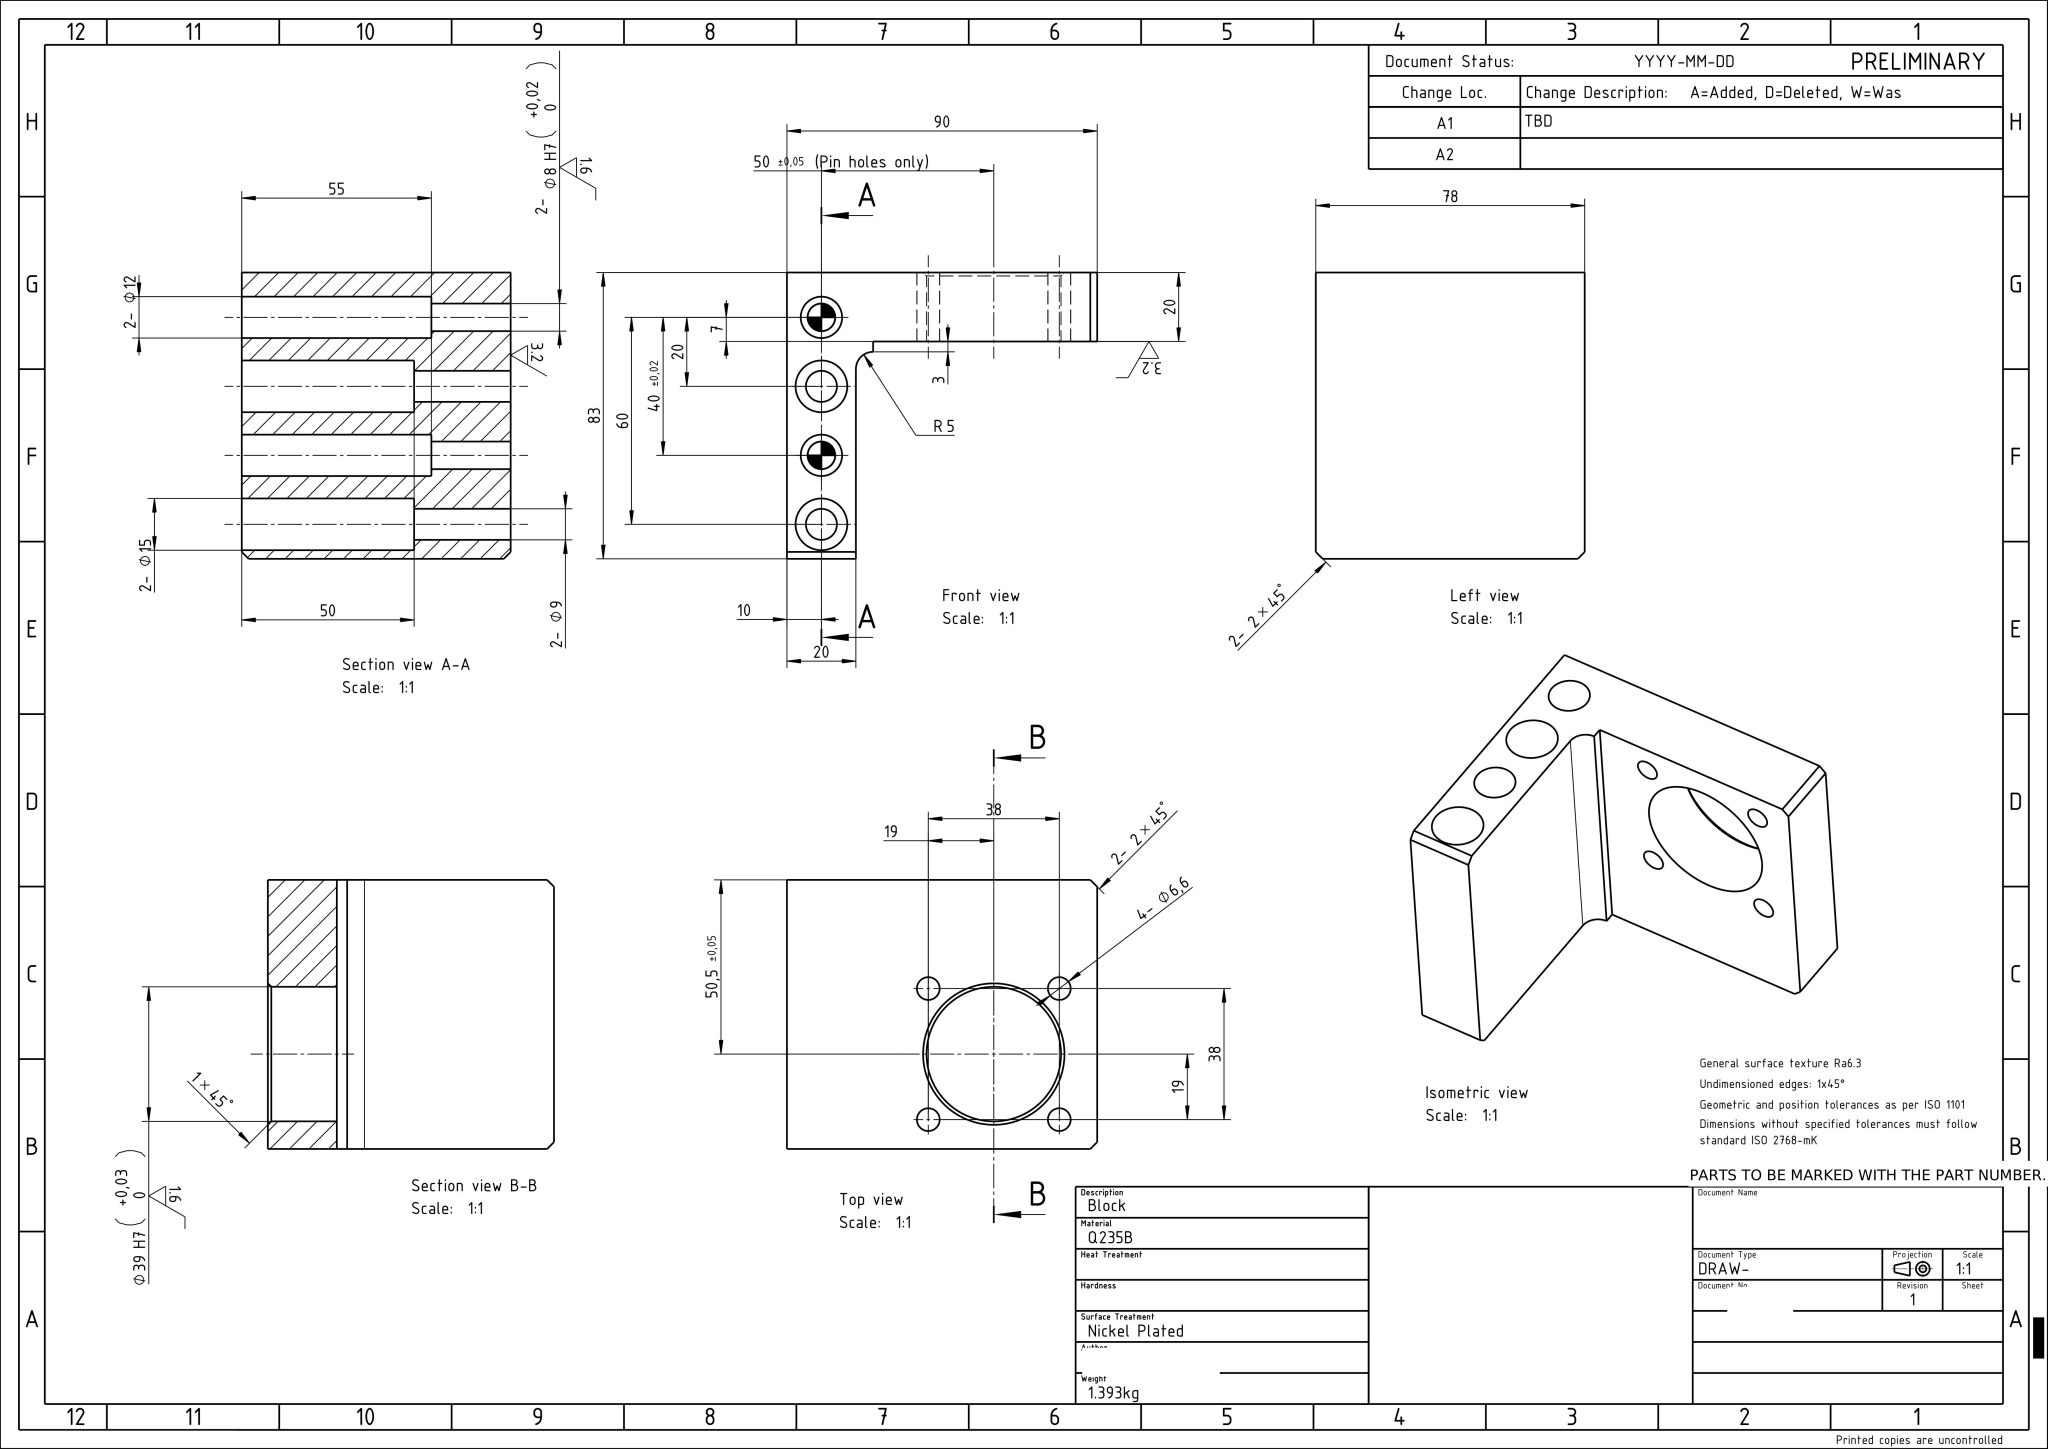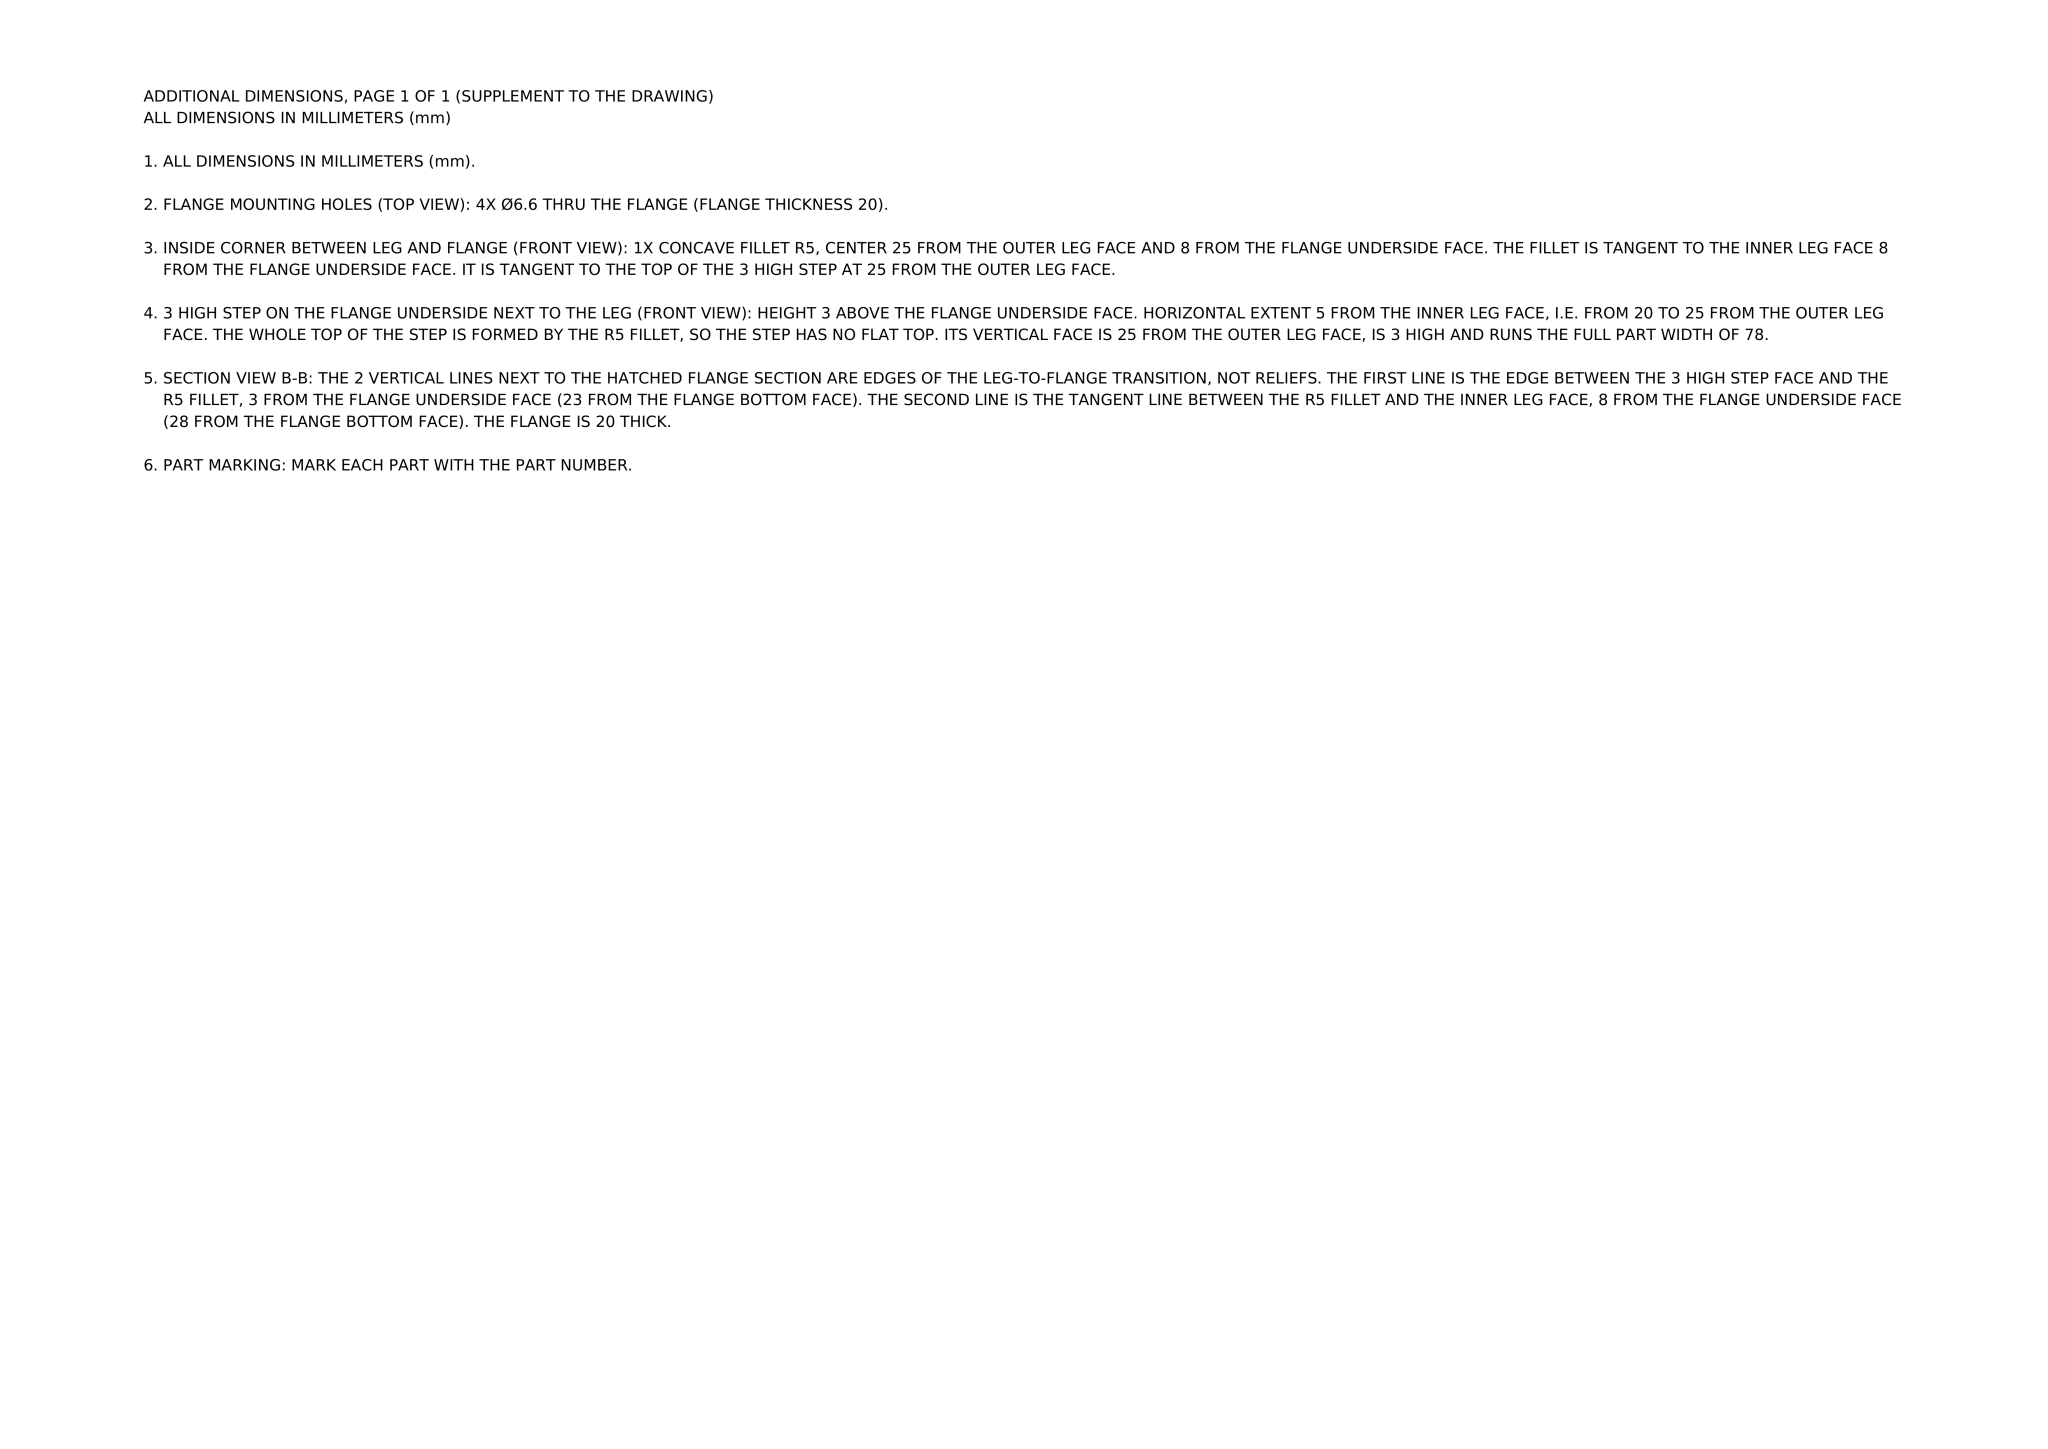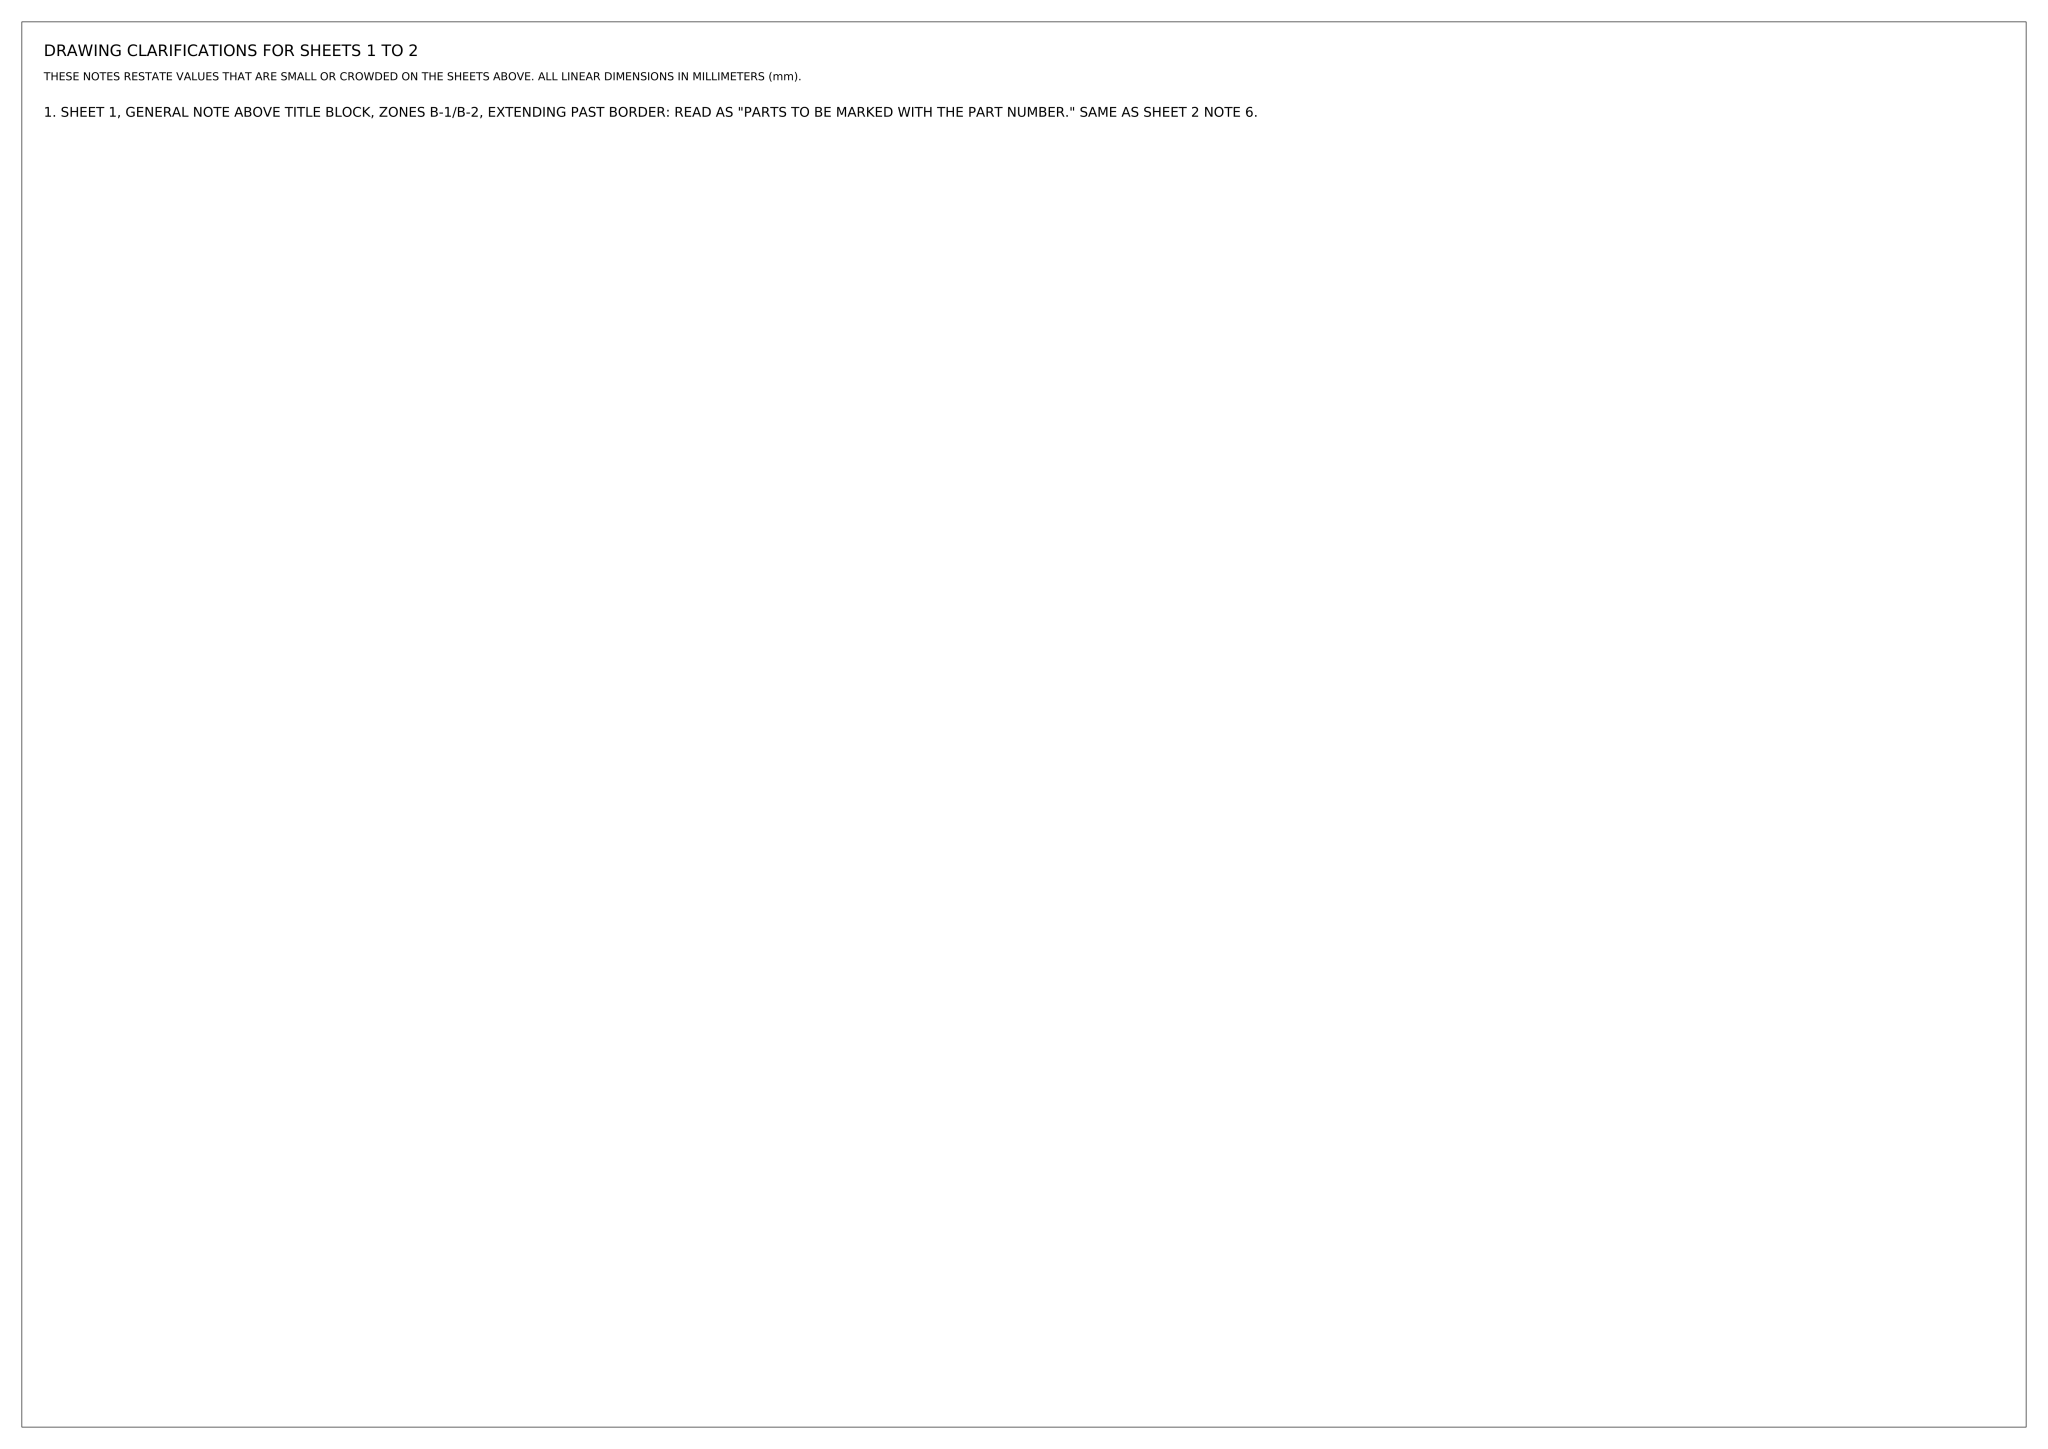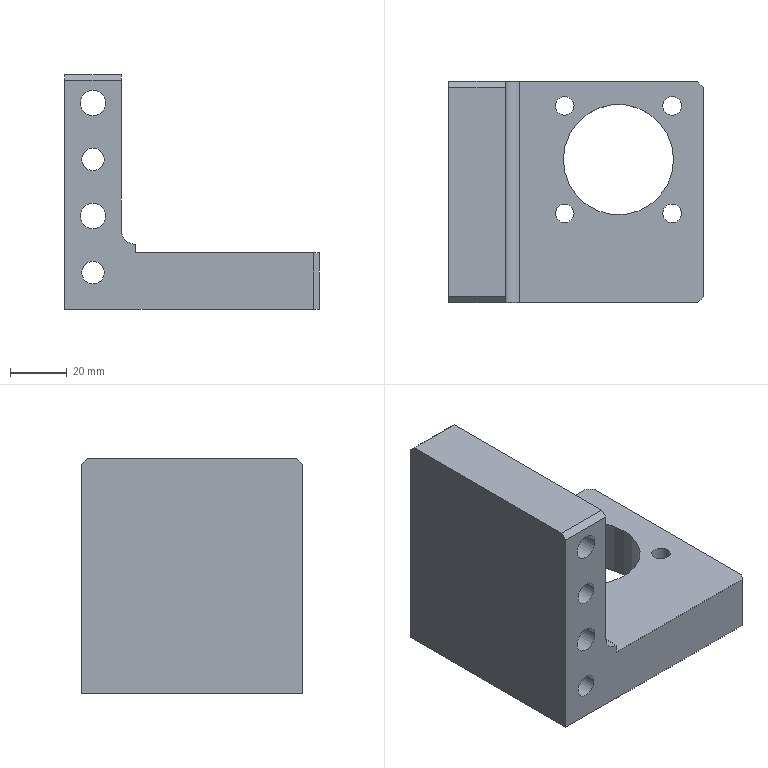Part | NX | mm | 1 solid | 32 faces | box 90 x 78 x 83 mm | volume 177430 mm3 | plane 17 | cylinder 14 | cone 1 | commonest cylinder face diameters 6.6 x4 8 x2 12 x2 9 x2 15 x2 10 x1 39 x1